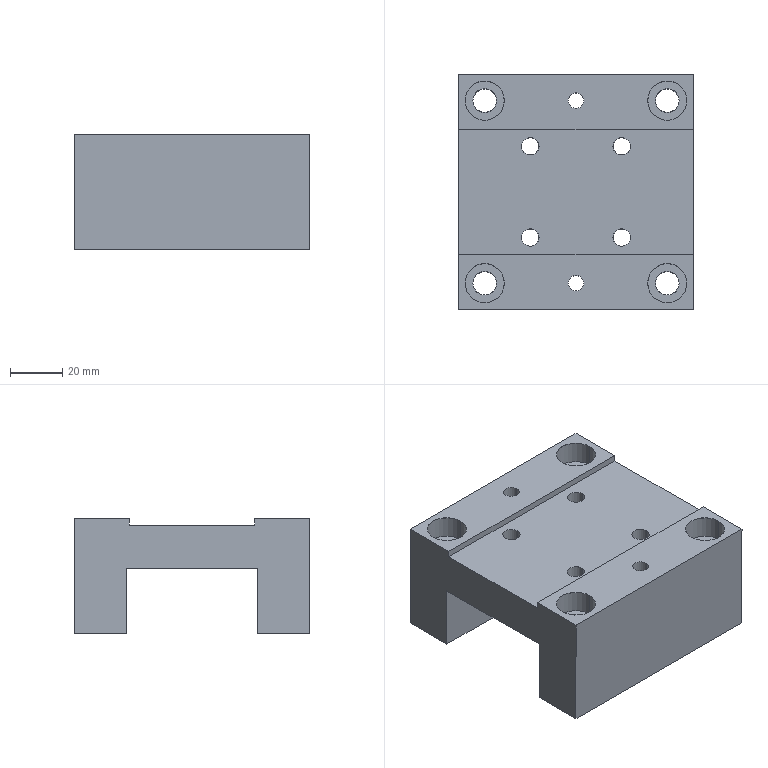Component | SolidWorks | X-AxisSliderRiserBlock-1 | 1 solid | 106 faces | box 90 x 90 x 44 mm | volume 211709 mm3 | cone 48 | cylinder 36 | plane 22 | commonest cylinder face diameters 15 x8 9 x8 11 x8 6.6 x8 6 x4
build123d program:
from build123d import *

# Parameters (mm, degrees)
SKETCH1_W                                      = 90
SKETCH1_H                                      = 90
BOSS_EXTRUDE1_DEPTH                            = 44
SKETCH2_W                                      = 90
SKETCH2_H                                      = 48
CUT_EXTRUDE1_DEPTH                             = 2.5
SKETCH9_W                                      = 50
SKETCH9_H                                      = 50
CUT_EXTRUDE2_DEPTH                             = 110.823
M6_HEX_SOCKET_HEAD_CAP_SCREW_CBORE1_AT_2_COUNT = 2
M6_HEX_SOCKET_HEAD_CAP_SCREW_CBORE1_AT_2_PITCH = 35
M6_HEX_SOCKET_HEAD_CAP_SCREW_CBORE1_AT_3_COUNT = 2
M6_HEX_SOCKET_HEAD_CAP_SCREW_CBORE1_AT_3_PITCH = 49.497
M6_HEX_SOCKET_HEAD_CAP_SCREW_CBORE1_AT_4_COUNT = 2
M6_HEX_SOCKET_HEAD_CAP_SCREW_CBORE1_AT_4_PITCH = 35
M8_HEX_SOCKET_HEAD_CAP_SCREW_CBORE1_AT_2_COUNT = 2
M8_HEX_SOCKET_HEAD_CAP_SCREW_CBORE1_AT_2_PITCH = 70
M8_HEX_SOCKET_HEAD_CAP_SCREW_CBORE1_AT_3_COUNT = 2
M8_HEX_SOCKET_HEAD_CAP_SCREW_CBORE1_AT_3_PITCH = 98.995
M8_HEX_SOCKET_HEAD_CAP_SCREW_CBORE1_AT_4_COUNT = 2
M8_HEX_SOCKET_HEAD_CAP_SCREW_CBORE1_AT_4_PITCH = 70
SKETCH6_R                                      = 3
CUT_EXTRUDE3_DEPTH                             = 78.369


with BuildPart() as part:
    # Sketch1 → Boss-Extrude1 (new body)
    with BuildSketch(Plane.XY):
        Rectangle(SKETCH1_W, SKETCH1_H)
    extrude(amount=BOSS_EXTRUDE1_DEPTH)

    # Sketch2 → Cut-Extrude1 (cut)
    with BuildSketch(Plane.XY.offset(44)):
        Rectangle(SKETCH2_W, SKETCH2_H)
    extrude(amount=-CUT_EXTRUDE1_DEPTH, mode=Mode.SUBTRACT)

    # Sketch9 → Cut-Extrude2 (cut, through all)
    with BuildSketch(Plane(origin=(45, 0, 0), x_dir=(0, 0, -1), z_dir=(1, 0, 0))):
        Rectangle(SKETCH9_W, SKETCH9_H)
    extrude(amount=-CUT_EXTRUDE2_DEPTH, mode=Mode.SUBTRACT)

    # Sketch4 → M6 Hex Socket Head Cap Screw CBORE1 (revolve, cut)
    with BuildSketch(Plane(origin=(17.5, 17.5, 25), x_dir=(0, 1, 0), z_dir=(1, 0, 0))):
        Polygon((0, 0), (0, 16.5), (3.325, 16.5), (3.3, 16.475), (3.3, 6.425), (3.325, 6.4), (5.5, 6.4), (5.5, 0.025), (5.525, 0), align=None)
    m6_hex_socket_head_cap_screw_cbore1 = revolve(axis=Axis((17.5, 17.5, 18.65), (0, 0, 1)), mode=Mode.SUBTRACT)

    # M6 Hex Socket Head Cap Screw CBORE1 at 2: M6 Hex Socket Head Cap Screw CBORE1 ×2
    with Locations(*[(-i * M6_HEX_SOCKET_HEAD_CAP_SCREW_CBORE1_AT_2_PITCH, 0, 0) for i in range(1, M6_HEX_SOCKET_HEAD_CAP_SCREW_CBORE1_AT_2_COUNT)]):
        add(m6_hex_socket_head_cap_screw_cbore1, mode=Mode.SUBTRACT)

    # M6 Hex Socket Head Cap Screw CBORE1 at 3: M6 Hex Socket Head Cap Screw CBORE1 ×2
    with Locations(*[Vector(-0.7071, -0.7071, 0) * (i * M6_HEX_SOCKET_HEAD_CAP_SCREW_CBORE1_AT_3_PITCH) for i in range(1, M6_HEX_SOCKET_HEAD_CAP_SCREW_CBORE1_AT_3_COUNT)]):
        add(m6_hex_socket_head_cap_screw_cbore1, mode=Mode.SUBTRACT)

    # M6 Hex Socket Head Cap Screw CBORE1 at 4: M6 Hex Socket Head Cap Screw CBORE1 ×2
    with Locations(*[(0, -i * M6_HEX_SOCKET_HEAD_CAP_SCREW_CBORE1_AT_4_PITCH, 0) for i in range(1, M6_HEX_SOCKET_HEAD_CAP_SCREW_CBORE1_AT_4_COUNT)]):
        add(m6_hex_socket_head_cap_screw_cbore1, mode=Mode.SUBTRACT)

    # Sketch7 → M8 Hex Socket Head Cap Screw CBORE1 (revolve, cut)
    with BuildSketch(Plane(origin=(-35, 35, 44), x_dir=(0, -1, 0), z_dir=(1, 0, 0))):
        Polygon((0, 0), (0, 44), (4.525, 44), (4.5, 43.975), (4.5, 8.625), (4.525, 8.6), (7.5, 8.6), (7.5, 0.025), (7.525, 0), align=None)
    m8_hex_socket_head_cap_screw_cbore1 = revolve(axis=Axis((-35, 35, 50.35), (0, 0, -1)), mode=Mode.SUBTRACT)

    # M8 Hex Socket Head Cap Screw CBORE1 at 2: M8 Hex Socket Head Cap Screw CBORE1 ×2
    with Locations(*[(i * M8_HEX_SOCKET_HEAD_CAP_SCREW_CBORE1_AT_2_PITCH, 0, 0) for i in range(1, M8_HEX_SOCKET_HEAD_CAP_SCREW_CBORE1_AT_2_COUNT)]):
        add(m8_hex_socket_head_cap_screw_cbore1, mode=Mode.SUBTRACT)

    # M8 Hex Socket Head Cap Screw CBORE1 at 3: M8 Hex Socket Head Cap Screw CBORE1 ×2
    with Locations(*[Vector(0.7071, -0.7071, 0) * (i * M8_HEX_SOCKET_HEAD_CAP_SCREW_CBORE1_AT_3_PITCH) for i in range(1, M8_HEX_SOCKET_HEAD_CAP_SCREW_CBORE1_AT_3_COUNT)]):
        add(m8_hex_socket_head_cap_screw_cbore1, mode=Mode.SUBTRACT)

    # M8 Hex Socket Head Cap Screw CBORE1 at 4: M8 Hex Socket Head Cap Screw CBORE1 ×2
    with Locations(*[(0, -i * M8_HEX_SOCKET_HEAD_CAP_SCREW_CBORE1_AT_4_PITCH, 0) for i in range(1, M8_HEX_SOCKET_HEAD_CAP_SCREW_CBORE1_AT_4_COUNT)]):
        add(m8_hex_socket_head_cap_screw_cbore1, mode=Mode.SUBTRACT)

    # Sketch6 → Cut-Extrude3 (cut, through all)
    with BuildSketch(Plane.XY.offset(44)):
        with Locations((0, 35)):
            Circle(SKETCH6_R)
        with Locations((0, -35)):
            Circle(SKETCH6_R)
    extrude(amount=-CUT_EXTRUDE3_DEPTH, mode=Mode.SUBTRACT)


solid = part.part

# Placed as in the assembly
solid = solid.moved(Location((19.229, -213.5, -12.5), (0, 0, 0)))